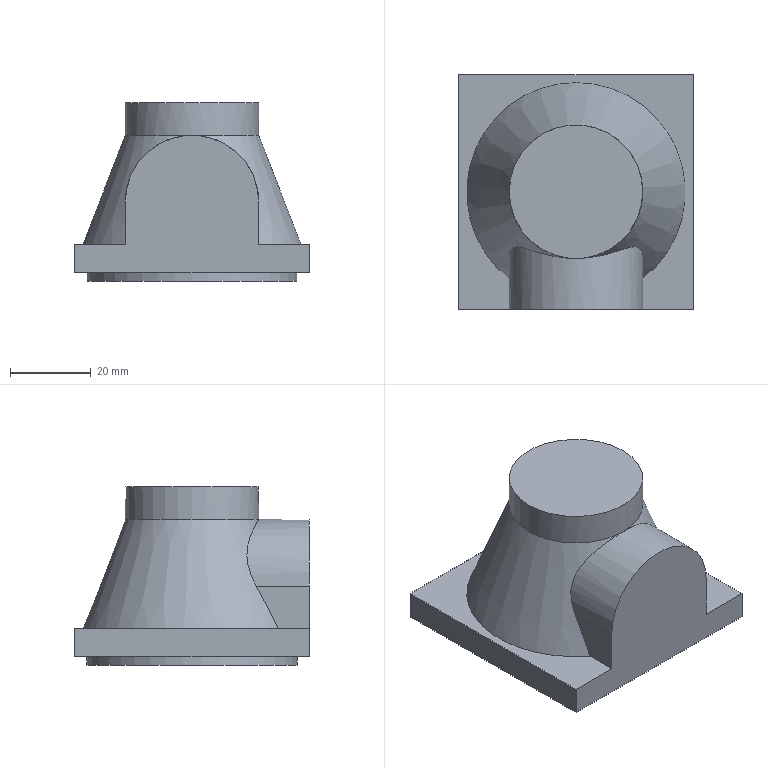CAM job | NX | mm | 3-axis | 1 set-up | 1 operations | part box 58 x 58 x 44
set-up 1
1. Cavity Milling | Mill Mill5 16 | CAVITY_MILL | path 51012.223 mm | 20.345 min